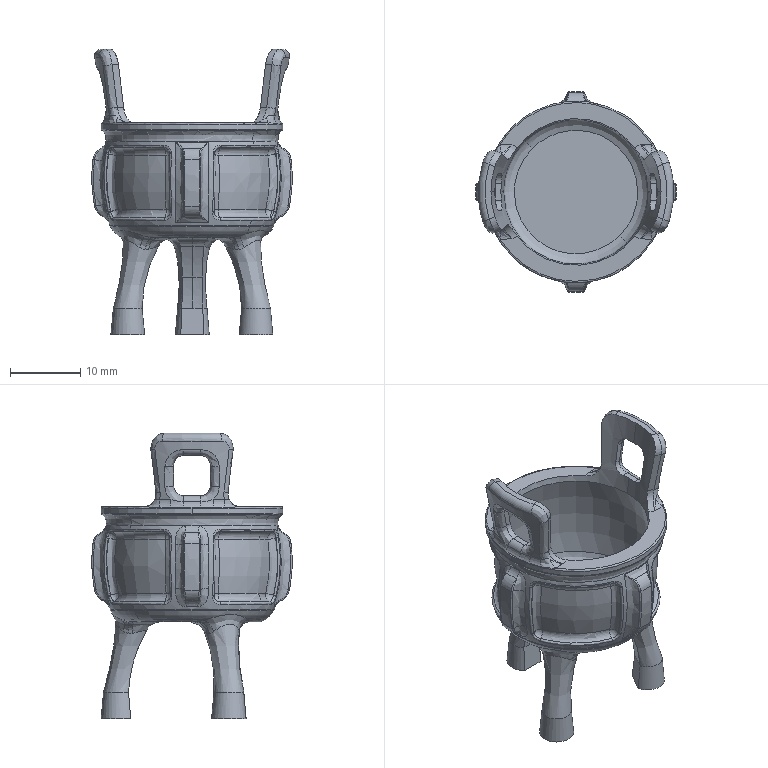CAM job | NX | mm | simultaneous | 1 set-up | 38 operations | part box 28.61 x 28.61 x 40.66
set-up 1
1. Cavity Milling | Mill Mill5 6 | CAVITY_MILL | path 10848.323 mm | 3.512 min
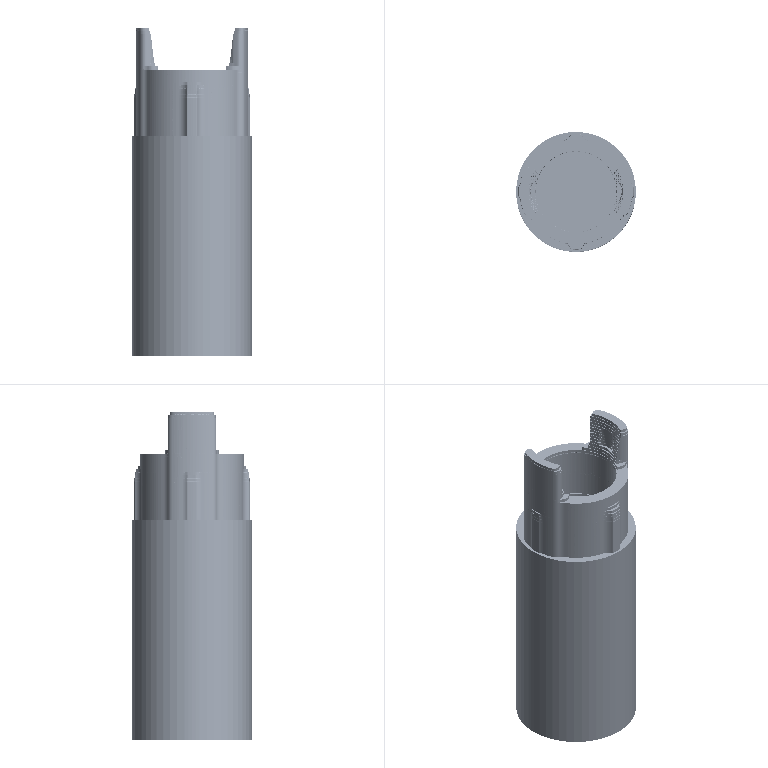2. Cavity Milling | Mill Mill5 4 | REST_MILLING_COPY | path 3792.271 mm | 2.924 min
3. Cavity Milling | Mill Mill5 4 | REST_MILLING_COPY_COPY | path 3664.236 mm | 2.848 min
4. Cavity Milling | Mill Mill5 2 | REST_MILLING_COPY_COPY_COPY | path 1356.59 mm | 1.515 min
5. Cavity Milling | Mill Mill5 2 | REST_MILLING_COPY_COPY_COPY_COPY | path 1125.005 mm | 1.245 min
6. Z-Level Milling | Mill Mill5 2 | ZLEVEL_PROFILE | path 46.217 mm | 0.03061 min
7. Z-Level Milling | Mill Mill5 2 | ZLEVEL_PROFILE_COPY | path 46.217 mm | 0.03061 min
8. Volume Based 2.5D Milling | Mill Mill5 6 | FLOOR_WALL | path 541.558 mm | 0.3839 min
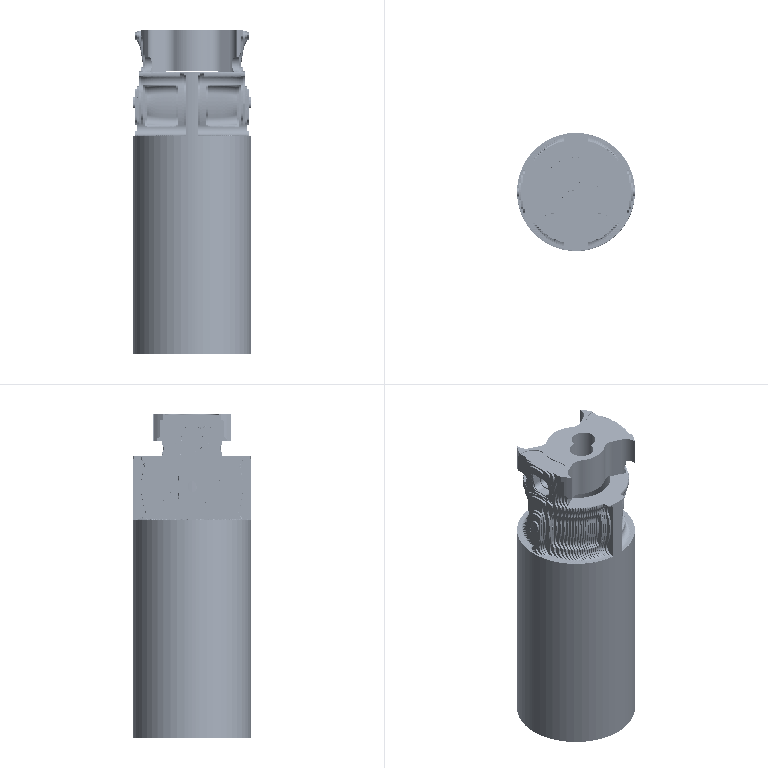9. Variable-axis Surface Contouring | Mill Mill5 6 | CONTOUR_PROFILE_COPY | path 83.568 mm | 0.0741 min
10. Variable-axis Surface Contouring | Mill Mill5 6 | CONTOUR_PROFILE | path 83.793 mm | 0.07438 min
11. Variable-axis Surface Contouring | Mill Mill5 R2 | VARIABLE_CONTOUR | path 6041.558 mm | 4.015 min
12. Fixed-axis Surface Contouring | Mill Mill5 R2 | CONTOUR_AREA | path 1122.053 mm | 0.7404 min
13. Fixed-axis Surface Contouring | Mill Mill5 R2 | CONTOUR_AREA_COPY_1 | path 1122.053 mm | 0.7404 min
14. Fixed-axis Surface Contouring | Mill Mill5 R1 | CONTOUR_AREA_COPY | path 2026.882 mm | 2.426 min
15. Fixed-axis Surface Contouring | Mill Mill5 R1 | CONTOUR_AREA_COPY_COPY | path 460.391 mm | 0.555 min
16. Fixed-axis Surface Contouring | Mill Mill5 R1 | CONTOUR_AREA_COPY_COPY_COPY | path 459.203 mm | 0.5503 min
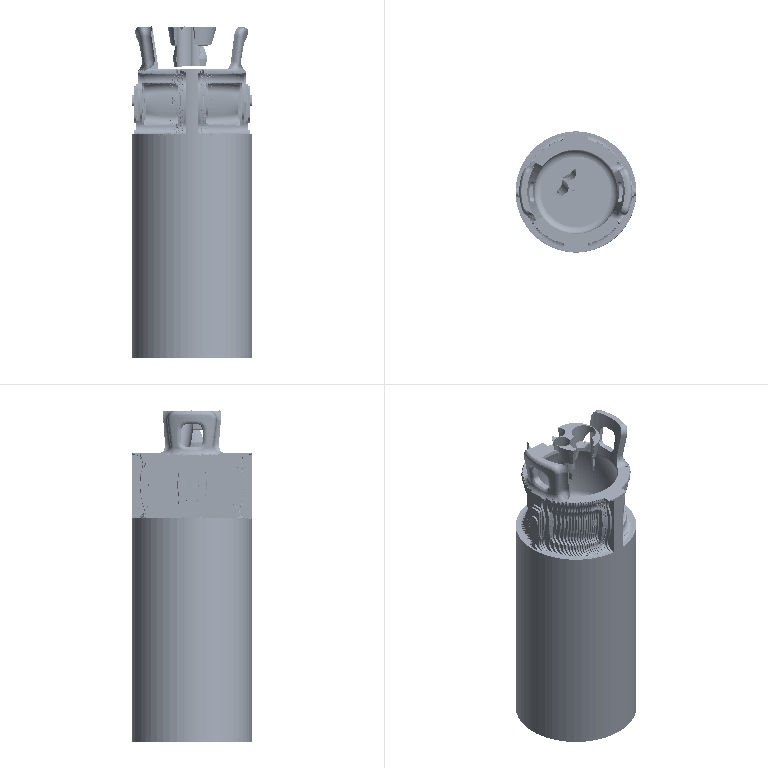17. Fixed-axis Surface Contouring | Mill Mill5 R1 | CONTOUR_AREA_COPY_COPY_1 | path 2026.882 mm | 2.426 min
18. Fixed-axis Surface Contouring | Mill Mill5 R1 | CONTOUR_AREA_COPY_COPY_COPY_1 | path 460.391 mm | 0.555 min
19. Fixed-axis Surface Contouring | Mill Mill5 R1 | CONTOUR_AREA_COPY_COPY_COPY_COPY | path 459.203 mm | 0.5503 min
20. Z-Level Milling | Mill Mill5 6 | ZLEVEL_PROFILE_1 | path 283.103 mm | 0.1109 min
21. Guided Curve Surface Contouring | Mill Mill5 R1 | VARIABLE_AXIS_GUIDING_CURVES_COPY_COPY_COPY | path 2292.753 mm | 2.761 min
22. Guided Curve Surface Contouring | Mill Mill5 R1 | VARIABLE_AXIS_GUIDING_CURVES_COPY_COPY_COPY_COPY_1 | path 2292.753 mm | 2.761 min
23. Guided Curve Surface Contouring | Mill Mill5 R1 | VARIABLE_AXIS_GUIDING_CURVES_COPY_COPY_COPY_COPY_COPY | path 8727.358 mm | 10.866 min
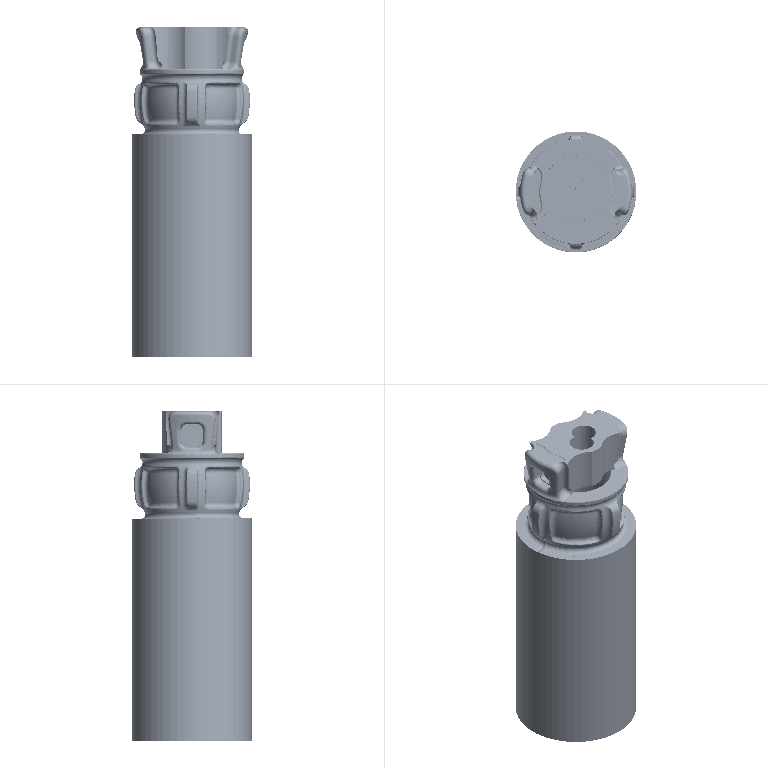24. Guided Curve Surface Contouring | Mill Mill5 R1 | VARIABLE_AXIS_GUIDING_CURVES_COPY_COPY_COPY_COPY | path 9009.714 mm | 11.219 min
25. Cavity Milling | Mill Mill5 6 | CAVITY_MILL_COPY | path 3494.547 mm | 1.118 min
26. Cavity Milling | Mill Mill5 6 | CAVITY_MILL_COPY_COPY | path 3529.509 mm | 1.126 min
27. Cavity Milling | Mill Mill5 6 | REST_MILLING_COPY_COPY_1 | path 4035.61 mm | 1.103 min
28. Z-Level Milling | Mill Mill5 4 | ZLEVEL_PROFILE_COPY_1 | path 354.917 mm | 0.155 min
29. Z-Level Milling | Mill Mill5 4 | ZLEVEL_PROFILE_COPY_1_COPY | path 354.917 mm | 0.155 min
30. Z-Level Milling | Mill Mill5 4 | ZLEVEL_PROFILE_COPY_1_COPY_1 | path 354.917 mm | 0.155 min
31. Guided Curve Surface Contouring | Mill Mill5 R2 | VARIABLE_AXIS_GUIDING_CURVES_1 | path 1332.45 mm | 0.8239 min
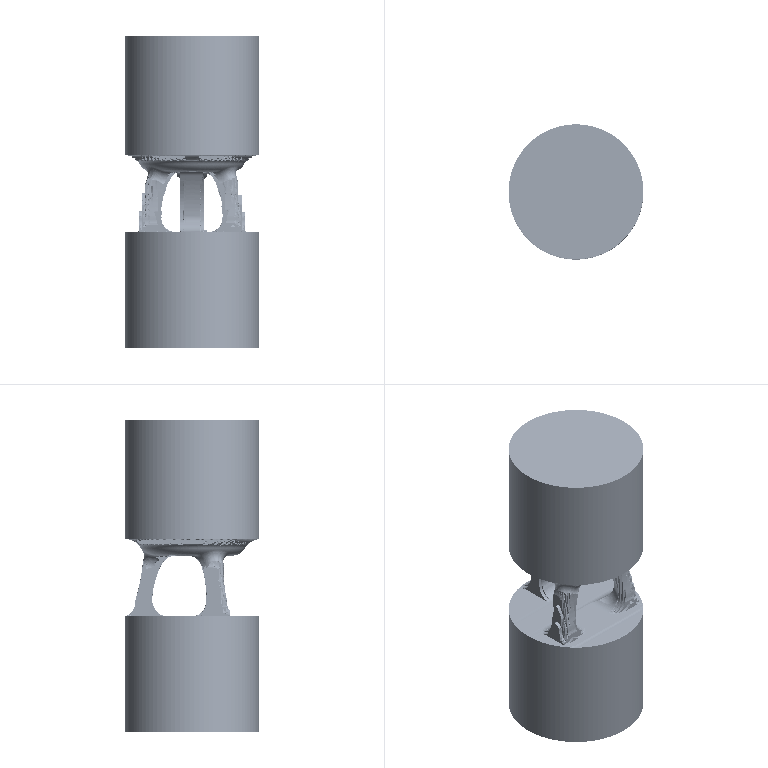32. Guided Curve Surface Contouring | Mill Mill5 R2 | VARIABLE_AXIS_GUIDING_CURVES_1_COPY_1_COPY_2 | path 1092.432 mm | 0.7094 min
33. Guided Curve Surface Contouring | Mill Mill5 R2 | VARIABLE_AXIS_GUIDING_CURVES_1_COPY_1_COPY_2_COPY | path 1092.432 mm | 0.7094 min
34. Guided Curve Surface Contouring | Mill Mill5 R2 | VARIABLE_AXIS_GUIDING_CURVES_1_COPY_1_COPY_2_COPY_1 | path 1092.432 mm | 0.7094 min
35. Guided Curve Surface Contouring | Mill Mill5 R2 | VARIABLE_AXIS_GUIDING_CURVES_1_COPY | path 375.905 mm | 0.2451 min
36. Guided Curve Surface Contouring | Mill Mill5 R2 | VARIABLE_AXIS_GUIDING_CURVES_1_COPY_COPY | path 375.905 mm | 0.2451 min
37. Guided Curve Surface Contouring | Mill Mill5 R2 | VARIABLE_AXIS_GUIDING_CURVES_1_COPY_COPY_1 | path 375.905 mm | 0.2451 min
38. Variable-axis Surface Contouring | Mill Mill5 6 | VARIABLE_STREAMLINE | path 1699.984 mm | 2.125 min